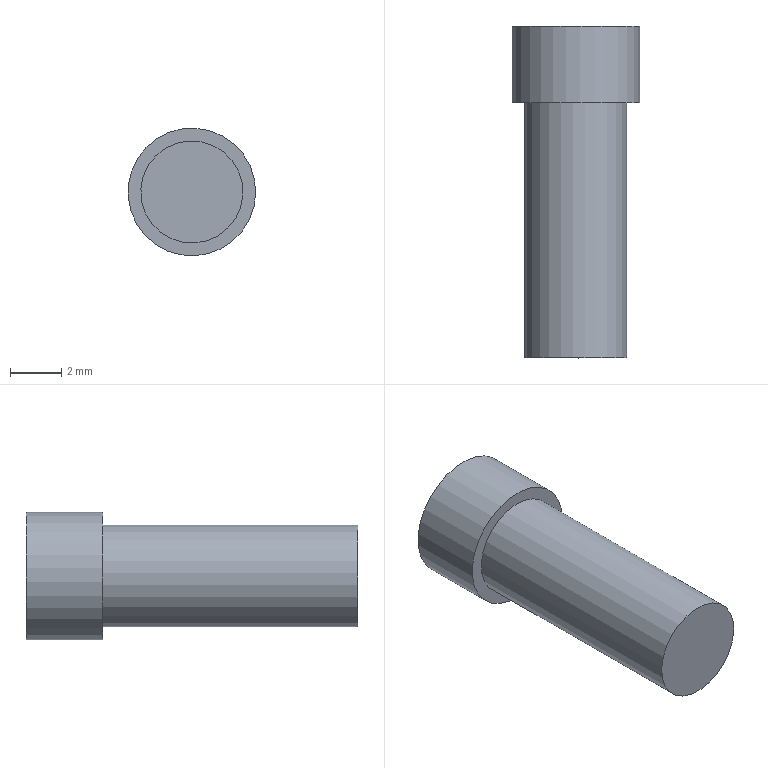Component | NX | SHEJI-WAIGUAN-4 | 1 solid | 5 faces | box 5 x 13 x 5 mm | volume 185 mm3 | plane 3 | cylinder 2 | commonest cylinder face diameters 4 x1 5 x1
STEP:
#1=CARTESIAN_POINT('',(0.,0.,0.));
#2=DIRECTION('',(0.,0.,1.));
#3=DIRECTION('',(1.,0.,0.));
#4=AXIS2_PLACEMENT_3D('',#1,#2,#3);
#5=CARTESIAN_POINT('',(-73.177,-5.,14.322));
#6=VERTEX_POINT('',#5);
#7=CARTESIAN_POINT('',(-75.,-5.,13.5));
#8=DIRECTION('',(0.,1.,0.));
#9=DIRECTION('',(0.9116,0.,0.4111));
#10=AXIS2_PLACEMENT_3D('',#7,#8,#9);
#11=CIRCLE('',#10,2.);
#12=CARTESIAN_POINT('',(-75.,-5.,13.5));
#13=DIRECTION('',(0.,-1.,0.));
#14=DIRECTION('',(0.9116,0.,0.4111));
#15=AXIS2_PLACEMENT_3D('',#12,#13,#14);
#16=PLANE('',#15);
#17=CARTESIAN_POINT('',(2.,0.));
#18=CARTESIAN_POINT('',(2.,-3.464));
#19=CARTESIAN_POINT('',(-1.,-1.732));
#20=CARTESIAN_POINT('',(-4.,-0.));
#21=CARTESIAN_POINT('',(-1.,1.732));
#22=CARTESIAN_POINT('',(2.,3.464));
#23=CARTESIAN_POINT('',(2.,0.));
#24=(BOUNDED_CURVE()B_SPLINE_CURVE(2,(#17,#18,#19,#20,#21,#22,#23),.UNSPECIFIED.,.T.,.F.)B_SPLINE_CURVE_WITH_KNOTS((1,2,2,2,2,1),(-2.094,0.,2.094,4.189,6.283,8.378),.UNSPECIFIED.)CURVE()GEOMETRIC_REPRESENTATION_ITEM()RATIONAL_B_SPLINE_CURVE((1.,0.5,1.,0.5,1.,0.5,1.))REPRESENTATION_ITEM(''));
#25=(GEOMETRIC_REPRESENTATION_CONTEXT(2)PARAMETRIC_REPRESENTATION_CONTEXT()REPRESENTATION_CONTEXT('',''));
#26=DEFINITIONAL_REPRESENTATION('',(#24),#25);
#27=PCURVE('',#16,#26);
#28=CARTESIAN_POINT('',(-75.,5.,13.5));
#29=DIRECTION('',(0.,-1.,0.));
#30=DIRECTION('',(0.9116,0.,0.4111));
#31=AXIS2_PLACEMENT_3D('',#28,#29,#30);
#32=CYLINDRICAL_SURFACE('',#31,2.);
#33=CARTESIAN_POINT('',(6.283,10.));
#34=DIRECTION('',(-1.,0.));
#35=VECTOR('',#34,1.);
#36=LINE('',#33,#35);
#37=(GEOMETRIC_REPRESENTATION_CONTEXT(2)PARAMETRIC_REPRESENTATION_CONTEXT()REPRESENTATION_CONTEXT('',''));
#38=DEFINITIONAL_REPRESENTATION('',(#36),#37);
#39=PCURVE('',#32,#38);
#40=SURFACE_CURVE('',#11,(#27,#39),.PCURVE_S1.);
#41=EDGE_CURVE('',#6,#6,#40,.T.);
#42=ORIENTED_EDGE('',*,*,#41,.F.);
#43=EDGE_LOOP('',(#42));
#44=FACE_BOUND('',#43,.T.);
#45=ADVANCED_FACE('',(#44),#16,.T.);
#46=ORIENTED_EDGE('',*,*,#41,.T.);
#47=CARTESIAN_POINT('',(-73.177,5.,14.322));
#48=VERTEX_POINT('',#47);
#49=CARTESIAN_POINT('',(-73.177,5.,14.322));
#50=CARTESIAN_POINT('',(-73.177,-5.,14.322));
#51=B_SPLINE_CURVE_WITH_KNOTS('',1,(#49,#50),.UNSPECIFIED.,.F.,.F.,(2,2),(0.,10.),.PIECEWISE_BEZIER_KNOTS.);
#52=CARTESIAN_POINT('',(0.,0.));
#53=DIRECTION('',(0.,1.));
#54=VECTOR('',#53,1.);
#55=LINE('',#52,#54);
#56=(GEOMETRIC_REPRESENTATION_CONTEXT(2)PARAMETRIC_REPRESENTATION_CONTEXT()REPRESENTATION_CONTEXT('',''));
#57=DEFINITIONAL_REPRESENTATION('',(#55),#56);
#58=PCURVE('',#32,#57);
#59=CARTESIAN_POINT('',(6.283,0.));
#60=DIRECTION('',(0.,1.));
#61=VECTOR('',#60,1.);
#62=LINE('',#59,#61);
#63=(GEOMETRIC_REPRESENTATION_CONTEXT(2)PARAMETRIC_REPRESENTATION_CONTEXT()REPRESENTATION_CONTEXT('',''));
#64=DEFINITIONAL_REPRESENTATION('',(#62),#63);
#65=PCURVE('',#32,#64);
#66=SEAM_CURVE('',#51,(#58,#65),.PCURVE_S1.);
#67=EDGE_CURVE('',#48,#6,#66,.T.);
#68=ORIENTED_EDGE('',*,*,#67,.F.);
#69=CARTESIAN_POINT('',(-75.,5.,13.5));
#70=DIRECTION('',(0.,-1.,0.));
#71=DIRECTION('',(0.9116,0.,0.4111));
#72=AXIS2_PLACEMENT_3D('',#69,#70,#71);
#73=CIRCLE('',#72,2.);
#74=CARTESIAN_POINT('',(0.,0.));
#75=DIRECTION('',(1.,0.));
#76=VECTOR('',#75,1.);
#77=LINE('',#74,#76);
#78=(GEOMETRIC_REPRESENTATION_CONTEXT(2)PARAMETRIC_REPRESENTATION_CONTEXT()REPRESENTATION_CONTEXT('',''));
#79=DEFINITIONAL_REPRESENTATION('',(#77),#78);
#80=PCURVE('',#32,#79);
#81=CARTESIAN_POINT('',(-75.,5.,13.5));
#82=DIRECTION('',(0.,-1.,0.));
#83=DIRECTION('',(0.9116,0.,0.4111));
#84=AXIS2_PLACEMENT_3D('',#81,#82,#83);
#85=PLANE('',#84);
#86=CARTESIAN_POINT('',(0.,0.));
#87=DIRECTION('',(1.,0.));
#88=AXIS2_PLACEMENT_2D('',#86,#87);
#89=CIRCLE('',#88,2.);
#90=(GEOMETRIC_REPRESENTATION_CONTEXT(2)PARAMETRIC_REPRESENTATION_CONTEXT()REPRESENTATION_CONTEXT('',''));
#91=DEFINITIONAL_REPRESENTATION('',(#89),#90);
#92=PCURVE('',#85,#91);
#93=SURFACE_CURVE('',#73,(#80,#92),.PCURVE_S1.);
#94=EDGE_CURVE('',#48,#48,#93,.T.);
#95=ORIENTED_EDGE('',*,*,#94,.T.);
#96=ORIENTED_EDGE('',*,*,#67,.T.);
#97=EDGE_LOOP('',(#46,#68,#95,#96));
#98=FACE_BOUND('',#97,.T.);
#99=ADVANCED_FACE('',(#98),#32,.T.);
#100=CARTESIAN_POINT('',(-72.721,8.,14.528));
#101=VERTEX_POINT('',#100);
#102=CARTESIAN_POINT('',(-75.,8.,13.5));
#103=DIRECTION('',(0.,-1.,0.));
#104=DIRECTION('',(0.9116,0.,0.4111));
#105=AXIS2_PLACEMENT_3D('',#102,#103,#104);
#106=CIRCLE('',#105,2.5);
#107=CARTESIAN_POINT('',(-75.,8.,13.5));
#108=DIRECTION('',(0.,1.,0.));
#109=DIRECTION('',(-0.9116,0.,-0.4111));
#110=AXIS2_PLACEMENT_3D('',#107,#108,#109);
#111=PLANE('',#110);
#112=CARTESIAN_POINT('',(-2.5,0.));
#113=CARTESIAN_POINT('',(-2.5,4.33));
#114=CARTESIAN_POINT('',(1.25,2.165));
#115=CARTESIAN_POINT('',(5.,-0.));
#116=CARTESIAN_POINT('',(1.25,-2.165));
#117=CARTESIAN_POINT('',(-2.5,-4.33));
#118=CARTESIAN_POINT('',(-2.5,0.));
#119=(BOUNDED_CURVE()B_SPLINE_CURVE(2,(#112,#113,#114,#115,#116,#117,#118),.UNSPECIFIED.,.T.,.F.)B_SPLINE_CURVE_WITH_KNOTS((1,2,2,2,2,1),(-2.094,0.,2.094,4.189,6.283,8.378),.UNSPECIFIED.)CURVE()GEOMETRIC_REPRESENTATION_ITEM()RATIONAL_B_SPLINE_CURVE((1.,0.5,1.,0.5,1.,0.5,1.))REPRESENTATION_ITEM(''));
#120=(GEOMETRIC_REPRESENTATION_CONTEXT(2)PARAMETRIC_REPRESENTATION_CONTEXT()REPRESENTATION_CONTEXT('',''));
#121=DEFINITIONAL_REPRESENTATION('',(#119),#120);
#122=PCURVE('',#111,#121);
#123=CARTESIAN_POINT('',(-75.,5.,13.5));
#124=DIRECTION('',(0.,1.,0.));
#125=DIRECTION('',(0.9116,0.,0.4111));
#126=AXIS2_PLACEMENT_3D('',#123,#124,#125);
#127=CYLINDRICAL_SURFACE('',#126,2.5);
#128=CARTESIAN_POINT('',(6.283,3.));
#129=DIRECTION('',(-1.,0.));
#130=VECTOR('',#129,1.);
#131=LINE('',#128,#130);
#132=(GEOMETRIC_REPRESENTATION_CONTEXT(2)PARAMETRIC_REPRESENTATION_CONTEXT()REPRESENTATION_CONTEXT('',''));
#133=DEFINITIONAL_REPRESENTATION('',(#131),#132);
#134=PCURVE('',#127,#133);
#135=SURFACE_CURVE('',#106,(#122,#134),.PCURVE_S1.);
#136=EDGE_CURVE('',#101,#101,#135,.T.);
#137=ORIENTED_EDGE('',*,*,#136,.F.);
#138=EDGE_LOOP('',(#137));
#139=FACE_BOUND('',#138,.T.);
#140=ADVANCED_FACE('',(#139),#111,.T.);
#141=ORIENTED_EDGE('',*,*,#94,.F.);
#142=EDGE_LOOP('',(#141));
#143=FACE_BOUND('',#142,.T.);
#144=CARTESIAN_POINT('',(-72.721,5.,14.528));
#145=VERTEX_POINT('',#144);
#146=CARTESIAN_POINT('',(-75.,5.,13.5));
#147=DIRECTION('',(0.,1.,0.));
#148=DIRECTION('',(0.9116,0.,0.4111));
#149=AXIS2_PLACEMENT_3D('',#146,#147,#148);
#150=CIRCLE('',#149,2.5);
#151=CARTESIAN_POINT('',(2.5,0.));
#152=CARTESIAN_POINT('',(2.5,-4.33));
#153=CARTESIAN_POINT('',(-1.25,-2.165));
#154=CARTESIAN_POINT('',(-5.,-0.));
#155=CARTESIAN_POINT('',(-1.25,2.165));
#156=CARTESIAN_POINT('',(2.5,4.33));
#157=CARTESIAN_POINT('',(2.5,0.));
#158=(BOUNDED_CURVE()B_SPLINE_CURVE(2,(#151,#152,#153,#154,#155,#156,#157),.UNSPECIFIED.,.T.,.F.)B_SPLINE_CURVE_WITH_KNOTS((1,2,2,2,2,1),(-2.094,0.,2.094,4.189,6.283,8.378),.UNSPECIFIED.)CURVE()GEOMETRIC_REPRESENTATION_ITEM()RATIONAL_B_SPLINE_CURVE((1.,0.5,1.,0.5,1.,0.5,1.))REPRESENTATION_ITEM(''));
#159=(GEOMETRIC_REPRESENTATION_CONTEXT(2)PARAMETRIC_REPRESENTATION_CONTEXT()REPRESENTATION_CONTEXT('',''));
#160=DEFINITIONAL_REPRESENTATION('',(#158),#159);
#161=PCURVE('',#85,#160);
#162=CARTESIAN_POINT('',(0.,0.));
#163=DIRECTION('',(1.,0.));
#164=VECTOR('',#163,1.);
#165=LINE('',#162,#164);
#166=(GEOMETRIC_REPRESENTATION_CONTEXT(2)PARAMETRIC_REPRESENTATION_CONTEXT()REPRESENTATION_CONTEXT('',''));
#167=DEFINITIONAL_REPRESENTATION('',(#165),#166);
#168=PCURVE('',#127,#167);
#169=SURFACE_CURVE('',#150,(#161,#168),.PCURVE_S1.);
#170=EDGE_CURVE('',#145,#145,#169,.T.);
#171=ORIENTED_EDGE('',*,*,#170,.F.);
#172=EDGE_LOOP('',(#171));
#173=FACE_BOUND('',#172,.T.);
#174=ADVANCED_FACE('',(#143,#173),#85,.T.);
#175=ORIENTED_EDGE('',*,*,#136,.T.);
#176=CARTESIAN_POINT('',(-72.721,5.,14.528));
#177=CARTESIAN_POINT('',(-72.721,8.,14.528));
#178=B_SPLINE_CURVE_WITH_KNOTS('',1,(#176,#177),.UNSPECIFIED.,.F.,.F.,(2,2),(0.,3.),.PIECEWISE_BEZIER_KNOTS.);
#179=CARTESIAN_POINT('',(0.,0.));
#180=DIRECTION('',(0.,1.));
#181=VECTOR('',#180,1.);
#182=LINE('',#179,#181);
#183=(GEOMETRIC_REPRESENTATION_CONTEXT(2)PARAMETRIC_REPRESENTATION_CONTEXT()REPRESENTATION_CONTEXT('',''));
#184=DEFINITIONAL_REPRESENTATION('',(#182),#183);
#185=PCURVE('',#127,#184);
#186=CARTESIAN_POINT('',(6.283,0.));
#187=DIRECTION('',(0.,1.));
#188=VECTOR('',#187,1.);
#189=LINE('',#186,#188);
#190=(GEOMETRIC_REPRESENTATION_CONTEXT(2)PARAMETRIC_REPRESENTATION_CONTEXT()REPRESENTATION_CONTEXT('',''));
#191=DEFINITIONAL_REPRESENTATION('',(#189),#190);
#192=PCURVE('',#127,#191);
#193=SEAM_CURVE('',#178,(#185,#192),.PCURVE_S1.);
#194=EDGE_CURVE('',#145,#101,#193,.T.);
#195=ORIENTED_EDGE('',*,*,#194,.F.);
#196=ORIENTED_EDGE('',*,*,#170,.T.);
#197=ORIENTED_EDGE('',*,*,#194,.T.);
#198=EDGE_LOOP('',(#175,#195,#196,#197));
#199=FACE_BOUND('',#198,.T.);
#200=ADVANCED_FACE('',(#199),#127,.T.);
#201=CLOSED_SHELL('',(#45,#99,#140,#174,#200));
#202=MANIFOLD_SOLID_BREP('',#201);
#203=(LENGTH_UNIT()NAMED_UNIT(*)SI_UNIT(.MILLI.,.METRE.));
#204=UNCERTAINTY_MEASURE_WITH_UNIT(LENGTH_MEASURE(0.00001),#203,'','');
#205=(NAMED_UNIT(*)PLANE_ANGLE_UNIT()SI_UNIT($,.RADIAN.));
#206=(NAMED_UNIT(*)SI_UNIT($,.STERADIAN.)SOLID_ANGLE_UNIT());
#207=(GEOMETRIC_REPRESENTATION_CONTEXT(3)GLOBAL_UNCERTAINTY_ASSIGNED_CONTEXT((#204))GLOBAL_UNIT_ASSIGNED_CONTEXT((#203,#205,#206))REPRESENTATION_CONTEXT('',''));
#208=ADVANCED_BREP_SHAPE_REPRESENTATION('',(#4,#202),#207);